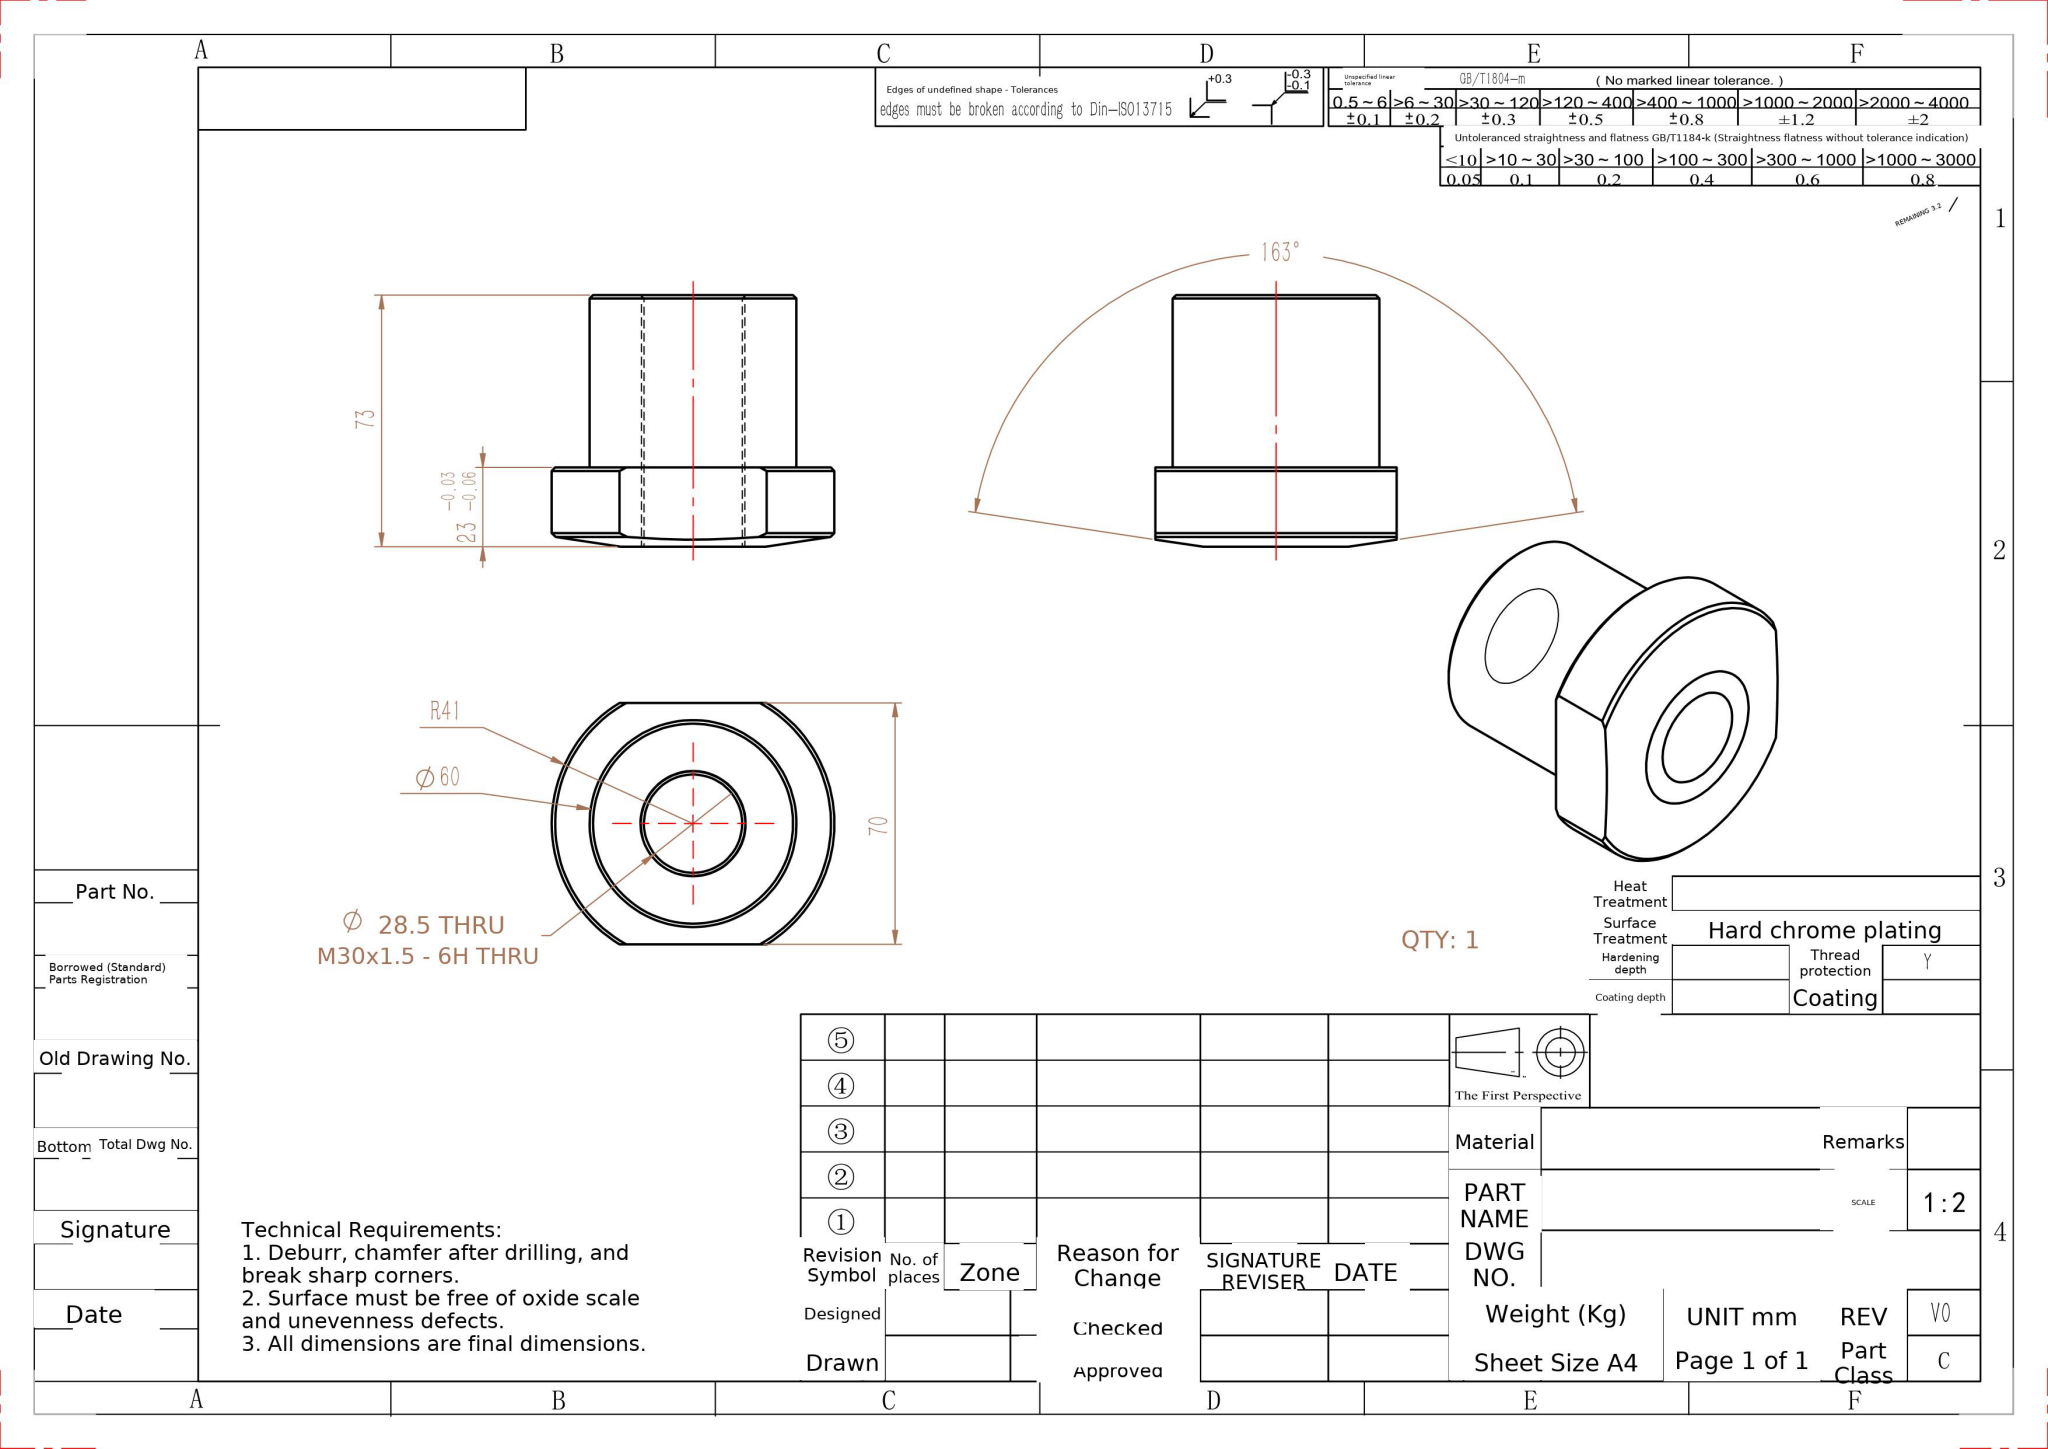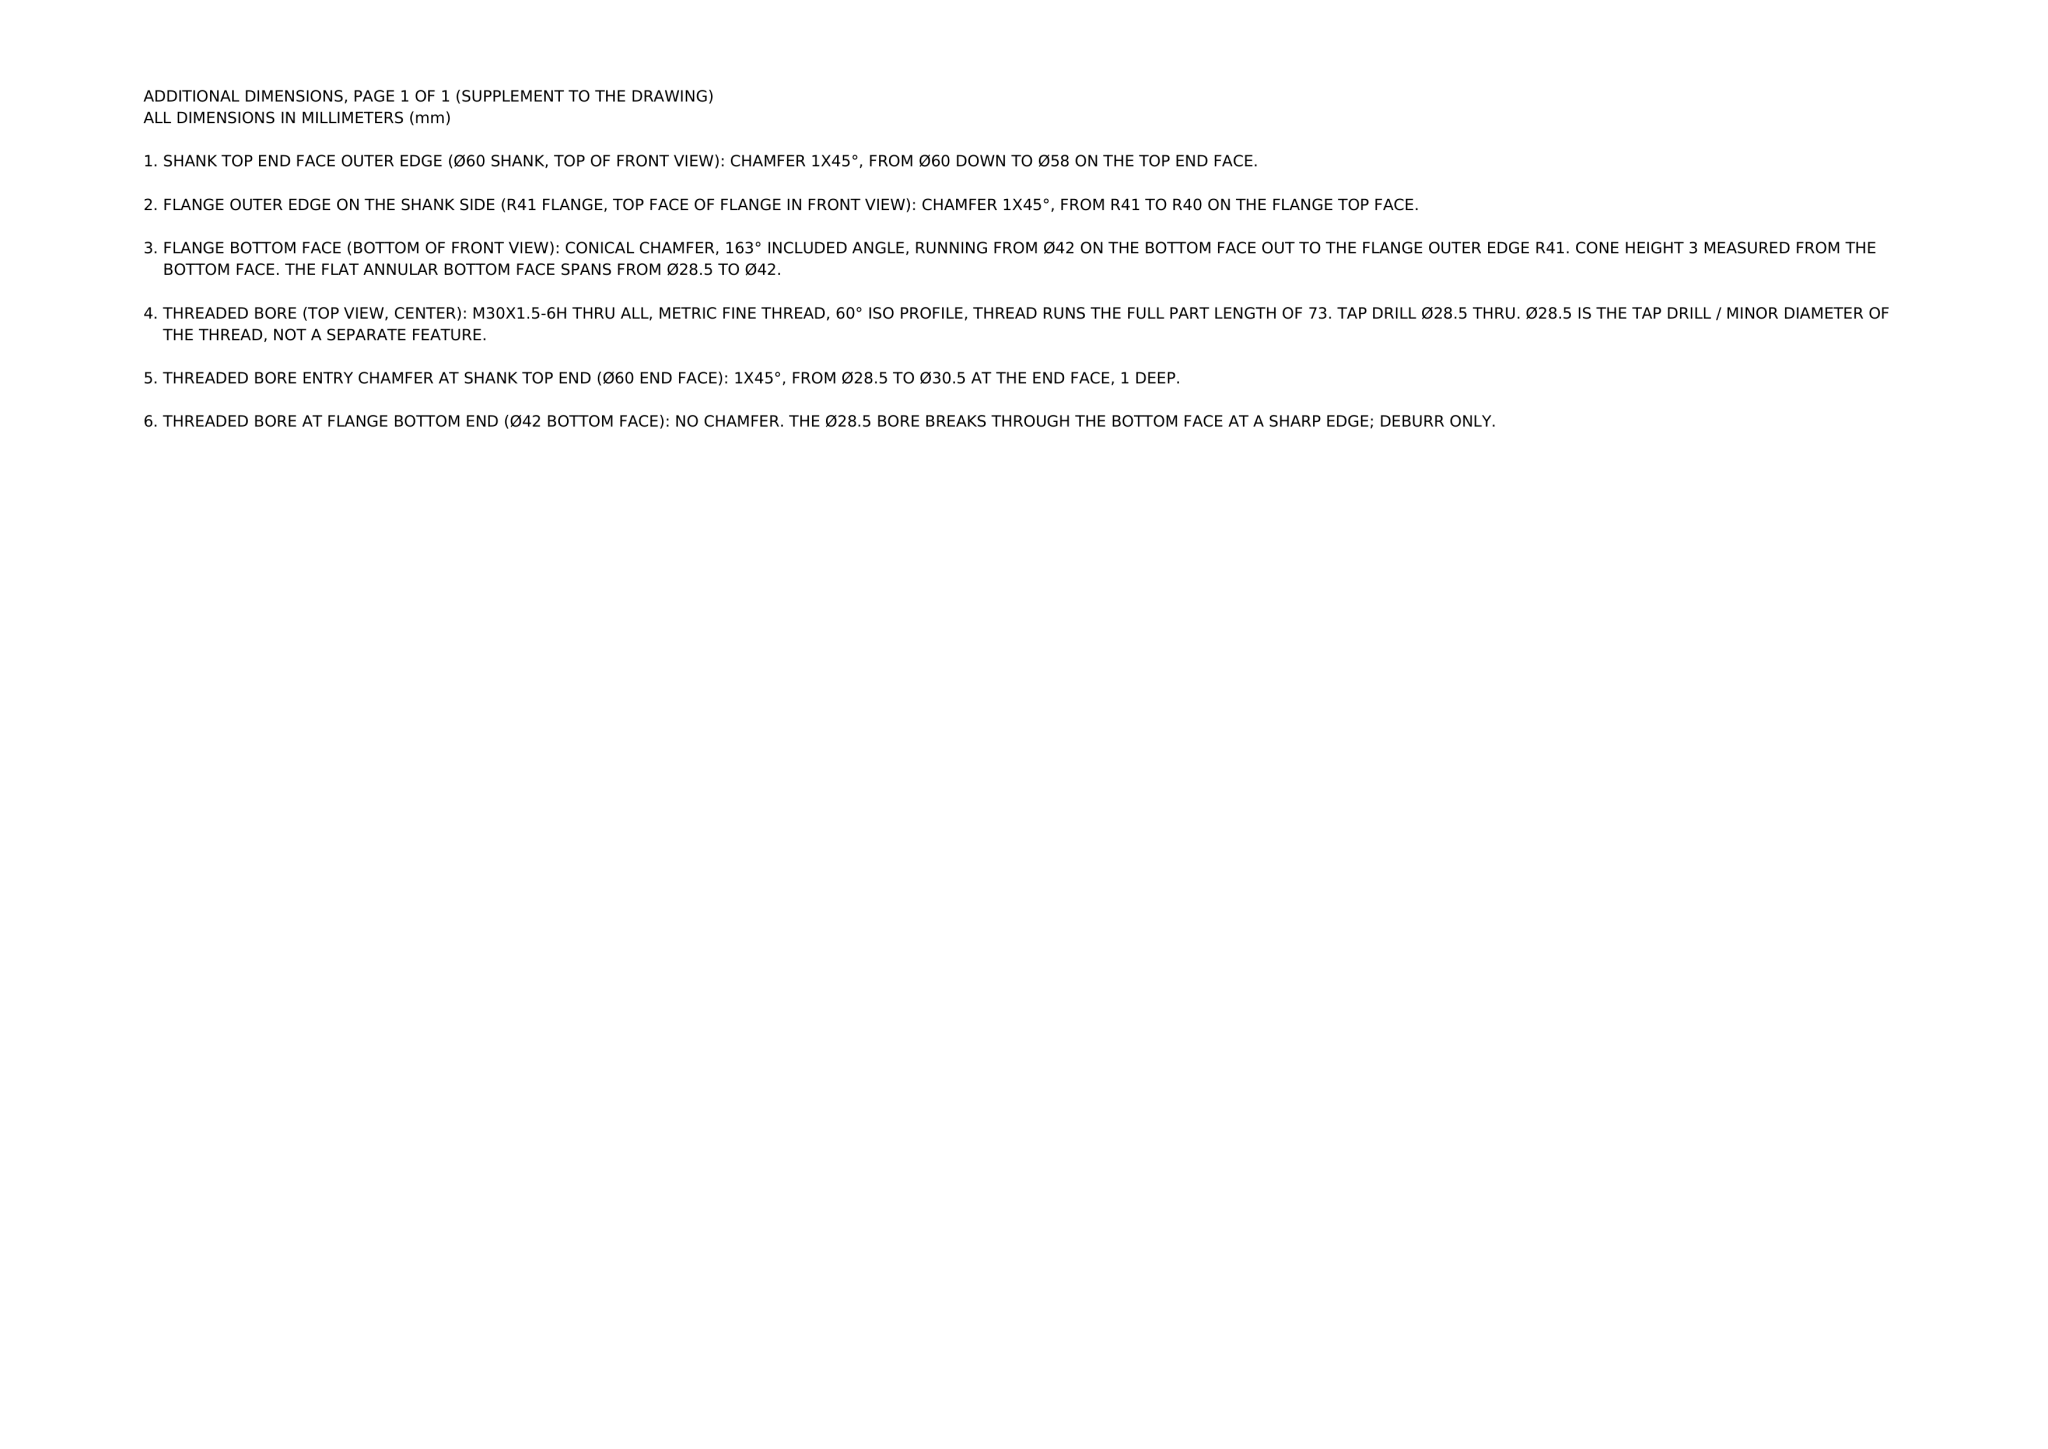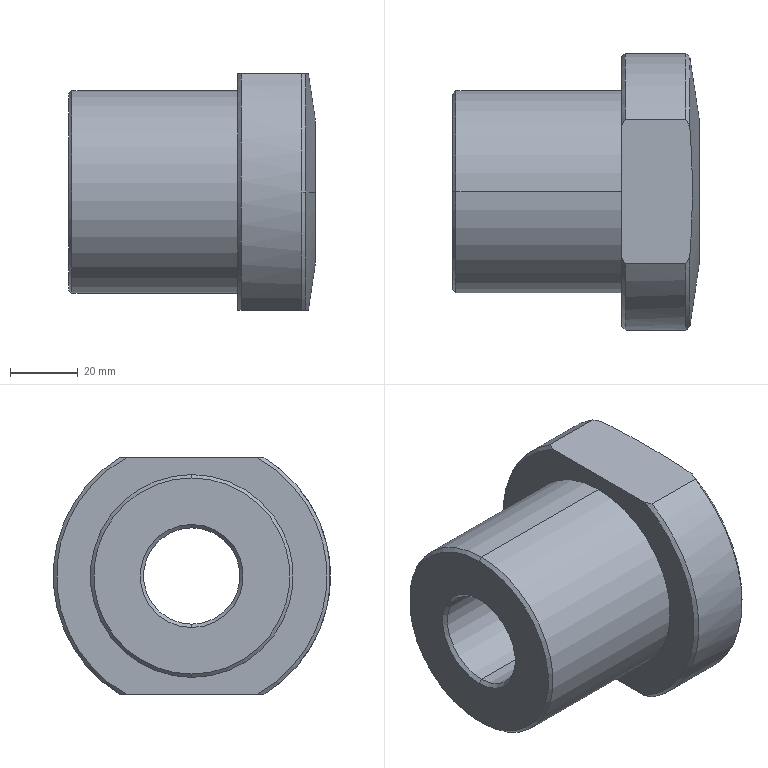Part | NX | mm | 1 solid | 22 faces | box 73 x 82 x 70 mm | volume 202408 mm3 | cone 11 | cylinder 6 | plane 5 | commonest cylinder face diameters 28.5 x2 60 x2 82 x2
STEP:
#1=CARTESIAN_POINT('',(23.176,-39.824,0.));
#2=VERTEX_POINT('',#1);
#3=CARTESIAN_POINT('',(23.176,-18.998,-35.));
#4=VERTEX_POINT('',#3);
#5=CARTESIAN_POINT('',(23.176,0.,0.));
#6=DIRECTION('',(1.,0.,0.));
#7=DIRECTION('',(-0.,1.,0.));
#8=AXIS2_PLACEMENT_3D('',#5,#6,#7);
#9=CIRCLE('',#8,39.824);
#10=EDGE_CURVE('',#2,#4,#9,.T.);
#11=ORIENTED_EDGE('',*,*,#10,.F.);
#12=CARTESIAN_POINT('',(22.,-41.,0.));
#13=VERTEX_POINT('',#12);
#14=CARTESIAN_POINT('',(23.176,-39.824,0.));
#15=DIRECTION('',(-0.7071,-0.7071,0.));
#16=VECTOR('',#15,1000.);
#17=LINE('',#14,#16);
#18=EDGE_CURVE('',#2,#13,#17,.T.);
#19=ORIENTED_EDGE('',*,*,#18,.T.);
#20=CARTESIAN_POINT('',(22.,-21.354,-35.));
#21=VERTEX_POINT('',#20);
#22=CARTESIAN_POINT('',(22.,0.,0.));
#23=DIRECTION('',(-1.,-0.,0.));
#24=DIRECTION('',(-0.,1.,0.));
#25=AXIS2_PLACEMENT_3D('',#22,#23,#24);
#26=CIRCLE('',#25,41.);
#27=EDGE_CURVE('',#21,#13,#26,.T.);
#28=ORIENTED_EDGE('',*,*,#27,.F.);
#29=CARTESIAN_POINT('',(23.176,-18.998,-35.));
#30=CARTESIAN_POINT('',(22.798,-19.79,-35.));
#31=CARTESIAN_POINT('',(22.406,-20.575,-35.));
#32=CARTESIAN_POINT('',(22.,-21.354,-35.));
#33=B_SPLINE_CURVE_WITH_KNOTS('',3,(#29,#30,#31,#32),.UNSPECIFIED.,.F.,.F.,(4,4),(0.,0.002634),.UNSPECIFIED.);
#34=EDGE_CURVE('',#4,#21,#33,.T.);
#35=ORIENTED_EDGE('',*,*,#34,.F.);
#36=EDGE_LOOP('',(#11,#19,#28,#35));
#37=FACE_OUTER_BOUND('',#36,.T.);
#38=CARTESIAN_POINT('',(23.176,0.,0.));
#39=DIRECTION('',(-1.,-0.,0.));
#40=DIRECTION('',(0.,-1.,0.));
#41=AXIS2_PLACEMENT_3D('',#38,#39,#40);
#42=CONICAL_SURFACE('',#41,39.824,0.7854);
#43=ADVANCED_FACE('',(#37),#42,.T.);
#44=CARTESIAN_POINT('',(-47.,0.,29.));
#45=VERTEX_POINT('',#44);
#46=CARTESIAN_POINT('',(-47.,0.,-29.));
#47=VERTEX_POINT('',#46);
#48=CARTESIAN_POINT('',(-47.,0.,0.));
#49=DIRECTION('',(-1.,0.,0.));
#50=DIRECTION('',(0.,0.,1.));
#51=AXIS2_PLACEMENT_3D('',#48,#49,#50);
#52=CIRCLE('',#51,29.);
#53=EDGE_CURVE('',#45,#47,#52,.T.);
#54=ORIENTED_EDGE('',*,*,#53,.F.);
#55=CARTESIAN_POINT('',(-46.,0.,30.));
#56=VERTEX_POINT('',#55);
#57=CARTESIAN_POINT('',(-47.,0.,29.));
#58=DIRECTION('',(0.7071,0.,0.7071));
#59=VECTOR('',#58,1000.);
#60=LINE('',#57,#59);
#61=EDGE_CURVE('',#45,#56,#60,.T.);
#62=ORIENTED_EDGE('',*,*,#61,.T.);
#63=CARTESIAN_POINT('',(-46.,0.,-30.));
#64=VERTEX_POINT('',#63);
#65=CARTESIAN_POINT('',(-46.,0.,0.));
#66=DIRECTION('',(1.,0.,0.));
#67=DIRECTION('',(0.,0.,1.));
#68=AXIS2_PLACEMENT_3D('',#65,#66,#67);
#69=CIRCLE('',#68,30.);
#70=EDGE_CURVE('',#64,#56,#69,.T.);
#71=ORIENTED_EDGE('',*,*,#70,.F.);
#72=CARTESIAN_POINT('',(-47.,0.,-29.));
#73=DIRECTION('',(0.7071,0.,-0.7071));
#74=VECTOR('',#73,1000.);
#75=LINE('',#72,#74);
#76=EDGE_CURVE('',#47,#64,#75,.T.);
#77=ORIENTED_EDGE('',*,*,#76,.F.);
#78=EDGE_LOOP('',(#54,#62,#71,#77));
#79=FACE_OUTER_BOUND('',#78,.T.);
#80=CARTESIAN_POINT('',(-47.,0.,0.));
#81=DIRECTION('',(1.,0.,0.));
#82=DIRECTION('',(0.,0.,-1.));
#83=AXIS2_PLACEMENT_3D('',#80,#81,#82);
#84=CONICAL_SURFACE('',#83,29.,0.7854);
#85=ADVANCED_FACE('',(#79),#84,.T.);
#86=CARTESIAN_POINT('',(-46.,0.,-14.25));
#87=VERTEX_POINT('',#86);
#88=CARTESIAN_POINT('',(-46.,0.,14.25));
#89=VERTEX_POINT('',#88);
#90=CARTESIAN_POINT('',(-46.,0.,0.));
#91=DIRECTION('',(-1.,0.,0.));
#92=DIRECTION('',(0.,0.,1.));
#93=AXIS2_PLACEMENT_3D('',#90,#91,#92);
#94=CIRCLE('',#93,14.25);
#95=EDGE_CURVE('',#87,#89,#94,.T.);
#96=ORIENTED_EDGE('',*,*,#95,.F.);
#97=CARTESIAN_POINT('',(-47.,0.,-15.25));
#98=VERTEX_POINT('',#97);
#99=CARTESIAN_POINT('',(-46.,0.,-14.25));
#100=DIRECTION('',(-0.7071,0.,-0.7071));
#101=VECTOR('',#100,1000.);
#102=LINE('',#99,#101);
#103=EDGE_CURVE('',#87,#98,#102,.T.);
#104=ORIENTED_EDGE('',*,*,#103,.T.);
#105=CARTESIAN_POINT('',(-47.,0.,15.25));
#106=VERTEX_POINT('',#105);
#107=CARTESIAN_POINT('',(-47.,0.,0.));
#108=DIRECTION('',(1.,0.,0.));
#109=DIRECTION('',(0.,0.,1.));
#110=AXIS2_PLACEMENT_3D('',#107,#108,#109);
#111=CIRCLE('',#110,15.25);
#112=EDGE_CURVE('',#106,#98,#111,.T.);
#113=ORIENTED_EDGE('',*,*,#112,.F.);
#114=CARTESIAN_POINT('',(-46.,0.,14.25));
#115=DIRECTION('',(-0.7071,0.,0.7071));
#116=VECTOR('',#115,1000.);
#117=LINE('',#114,#116);
#118=EDGE_CURVE('',#89,#106,#117,.T.);
#119=ORIENTED_EDGE('',*,*,#118,.F.);
#120=EDGE_LOOP('',(#96,#104,#113,#119));
#121=FACE_OUTER_BOUND('',#120,.T.);
#122=CARTESIAN_POINT('',(-46.,0.,0.));
#123=DIRECTION('',(-1.,0.,0.));
#124=DIRECTION('',(0.,0.,1.));
#125=AXIS2_PLACEMENT_3D('',#122,#123,#124);
#126=CONICAL_SURFACE('',#125,14.25,0.7854);
#127=ADVANCED_FACE('',(#121),#126,.F.);
#128=CARTESIAN_POINT('',(26.,0.,-14.25));
#129=VERTEX_POINT('',#128);
#130=CARTESIAN_POINT('',(26.,0.,14.25));
#131=VERTEX_POINT('',#130);
#132=CARTESIAN_POINT('',(26.,0.,0.));
#133=DIRECTION('',(-1.,0.,0.));
#134=DIRECTION('',(0.,0.,1.));
#135=AXIS2_PLACEMENT_3D('',#132,#133,#134);
#136=CIRCLE('',#135,14.25);
#137=EDGE_CURVE('',#129,#131,#136,.T.);
#138=ORIENTED_EDGE('',*,*,#137,.F.);
#139=CARTESIAN_POINT('',(-47.,0.,-14.25));
#140=DIRECTION('',(-1.,0.,0.));
#141=VECTOR('',#140,1000.);
#142=LINE('',#139,#141);
#143=EDGE_CURVE('',#129,#87,#142,.T.);
#144=ORIENTED_EDGE('',*,*,#143,.T.);
#145=ORIENTED_EDGE('',*,*,#95,.T.);
#146=CARTESIAN_POINT('',(-47.,0.,14.25));
#147=DIRECTION('',(-1.,0.,0.));
#148=VECTOR('',#147,1000.);
#149=LINE('',#146,#148);
#150=EDGE_CURVE('',#131,#89,#149,.T.);
#151=ORIENTED_EDGE('',*,*,#150,.F.);
#152=EDGE_LOOP('',(#138,#144,#145,#151));
#153=FACE_OUTER_BOUND('',#152,.T.);
#154=CARTESIAN_POINT('',(-47.,0.,0.));
#155=DIRECTION('',(-1.,0.,0.));
#156=DIRECTION('',(0.,0.,1.));
#157=AXIS2_PLACEMENT_3D('',#154,#155,#156);
#158=CYLINDRICAL_SURFACE('',#157,14.25);
#159=ADVANCED_FACE('',(#153),#158,.F.);
#160=ORIENTED_EDGE('',*,*,#70,.T.);
#161=CARTESIAN_POINT('',(3.,0.,30.));
#162=VERTEX_POINT('',#161);
#163=CARTESIAN_POINT('',(-47.,0.,30.));
#164=DIRECTION('',(1.,0.,0.));
#165=VECTOR('',#164,1000.);
#166=LINE('',#163,#165);
#167=EDGE_CURVE('',#56,#162,#166,.T.);
#168=ORIENTED_EDGE('',*,*,#167,.T.);
#169=CARTESIAN_POINT('',(3.,0.,-30.));
#170=VERTEX_POINT('',#169);
#171=CARTESIAN_POINT('',(3.,0.,0.));
#172=DIRECTION('',(-1.,0.,0.));
#173=DIRECTION('',(0.,0.,1.));
#174=AXIS2_PLACEMENT_3D('',#171,#172,#173);
#175=CIRCLE('',#174,30.);
#176=EDGE_CURVE('',#162,#170,#175,.T.);
#177=ORIENTED_EDGE('',*,*,#176,.T.);
#178=CARTESIAN_POINT('',(-47.,0.,-30.));
#179=DIRECTION('',(1.,0.,0.));
#180=VECTOR('',#179,1000.);
#181=LINE('',#178,#180);
#182=EDGE_CURVE('',#64,#170,#181,.T.);
#183=ORIENTED_EDGE('',*,*,#182,.F.);
#184=EDGE_LOOP('',(#160,#168,#177,#183));
#185=FACE_OUTER_BOUND('',#184,.T.);
#186=CARTESIAN_POINT('',(-47.,0.,0.));
#187=DIRECTION('',(1.,0.,0.));
#188=DIRECTION('',(0.,0.,-1.));
#189=AXIS2_PLACEMENT_3D('',#186,#187,#188);
#190=CYLINDRICAL_SURFACE('',#189,30.);
#191=ADVANCED_FACE('',(#185),#190,.T.);
#192=CARTESIAN_POINT('',(26.,21.,0.));
#193=VERTEX_POINT('',#192);
#194=CARTESIAN_POINT('',(26.,-21.,0.));
#195=VERTEX_POINT('',#194);
#196=CARTESIAN_POINT('',(26.,0.,0.));
#197=DIRECTION('',(1.,0.,0.));
#198=DIRECTION('',(-0.,1.,0.));
#199=AXIS2_PLACEMENT_3D('',#196,#197,#198);
#200=CIRCLE('',#199,21.);
#201=EDGE_CURVE('',#193,#195,#200,.T.);
#202=ORIENTED_EDGE('',*,*,#201,.F.);
#203=CARTESIAN_POINT('',(23.176,39.824,0.));
#204=VERTEX_POINT('',#203);
#205=CARTESIAN_POINT('',(26.,21.,0.));
#206=DIRECTION('',(-0.1483,0.9889,0.));
#207=VECTOR('',#206,1000.);
#208=LINE('',#205,#207);
#209=EDGE_CURVE('',#193,#204,#208,.T.);
#210=ORIENTED_EDGE('',*,*,#209,.T.);
#211=CARTESIAN_POINT('',(23.176,18.998,35.));
#212=VERTEX_POINT('',#211);
#213=CARTESIAN_POINT('',(23.176,0.,0.));
#214=DIRECTION('',(1.,0.,0.));
#215=DIRECTION('',(-0.,1.,0.));
#216=AXIS2_PLACEMENT_3D('',#213,#214,#215);
#217=CIRCLE('',#216,39.824);
#218=EDGE_CURVE('',#204,#212,#217,.T.);
#219=ORIENTED_EDGE('',*,*,#218,.T.);
#220=CARTESIAN_POINT('',(23.176,-18.998,35.));
#221=VERTEX_POINT('',#220);
#222=CARTESIAN_POINT('',(23.176,18.998,35.));
#223=CARTESIAN_POINT('',(23.402,15.846,35.));
#224=CARTESIAN_POINT('',(23.584,12.691,35.));
#225=CARTESIAN_POINT('',(23.833,6.372,35.));
#226=CARTESIAN_POINT('',(23.899,3.208,35.));
#227=CARTESIAN_POINT('',(23.901,-3.129,35.));
#228=CARTESIAN_POINT('',(23.835,-6.303,35.));
#229=CARTESIAN_POINT('',(23.586,-12.659,35.));
#230=CARTESIAN_POINT('',(23.403,-15.83,35.));
#231=CARTESIAN_POINT('',(23.176,-18.998,35.));
#232=B_SPLINE_CURVE_WITH_KNOTS('',3,(#222,#223,#224,#225,#226,#227,#228,#229,#230,#231),.UNSPECIFIED.,.F.,.F.,(4,2,2,2,4),(0.04542,0.0549,0.06438,0.07386,0.08334),.UNSPECIFIED.);
#233=EDGE_CURVE('',#212,#221,#232,.T.);
#234=ORIENTED_EDGE('',*,*,#233,.T.);
#235=CARTESIAN_POINT('',(23.176,0.,0.));
#236=DIRECTION('',(1.,0.,0.));
#237=DIRECTION('',(-0.,1.,0.));
#238=AXIS2_PLACEMENT_3D('',#235,#236,#237);
#239=CIRCLE('',#238,39.824);
#240=EDGE_CURVE('',#221,#2,#239,.T.);
#241=ORIENTED_EDGE('',*,*,#240,.T.);
#242=CARTESIAN_POINT('',(26.,-21.,0.));
#243=DIRECTION('',(-0.1483,-0.9889,0.));
#244=VECTOR('',#243,1000.);
#245=LINE('',#242,#244);
#246=EDGE_CURVE('',#195,#2,#245,.T.);
#247=ORIENTED_EDGE('',*,*,#246,.F.);
#248=EDGE_LOOP('',(#202,#210,#219,#234,#241,#247));
#249=FACE_OUTER_BOUND('',#248,.T.);
#250=CARTESIAN_POINT('',(26.,0.,0.));
#251=DIRECTION('',(-1.,-0.,0.));
#252=DIRECTION('',(0.,-1.,0.));
#253=AXIS2_PLACEMENT_3D('',#250,#251,#252);
#254=CONICAL_SURFACE('',#253,21.,1.422);
#255=ADVANCED_FACE('',(#249),#254,.T.);
#256=CARTESIAN_POINT('',(22.,21.354,35.));
#257=VERTEX_POINT('',#256);
#258=CARTESIAN_POINT('',(4.,21.354,35.));
#259=VERTEX_POINT('',#258);
#260=CARTESIAN_POINT('',(141.966,21.354,35.));
#261=DIRECTION('',(-1.,0.,0.));
#262=VECTOR('',#261,1000.);
#263=LINE('',#260,#262);
#264=EDGE_CURVE('',#257,#259,#263,.T.);
#265=ORIENTED_EDGE('',*,*,#264,.F.);
#266=CARTESIAN_POINT('',(22.,21.354,-35.));
#267=VERTEX_POINT('',#266);
#268=CARTESIAN_POINT('',(22.,0.,0.));
#269=DIRECTION('',(-1.,-0.,0.));
#270=DIRECTION('',(-0.,1.,0.));
#271=AXIS2_PLACEMENT_3D('',#268,#269,#270);
#272=CIRCLE('',#271,41.);
#273=EDGE_CURVE('',#257,#267,#272,.T.);
#274=ORIENTED_EDGE('',*,*,#273,.T.);
#275=CARTESIAN_POINT('',(4.,21.354,-35.));
#276=VERTEX_POINT('',#275);
#277=CARTESIAN_POINT('',(141.966,21.354,-35.));
#278=DIRECTION('',(1.,0.,0.));
#279=VECTOR('',#278,1000.);
#280=LINE('',#277,#279);
#281=EDGE_CURVE('',#276,#267,#280,.T.);
#282=ORIENTED_EDGE('',*,*,#281,.F.);
#283=CARTESIAN_POINT('',(4.,0.,0.));
#284=DIRECTION('',(1.,0.,0.));
#285=DIRECTION('',(0.,-0.,1.));
#286=AXIS2_PLACEMENT_3D('',#283,#284,#285);
#287=CIRCLE('',#286,41.);
#288=EDGE_CURVE('',#276,#259,#287,.T.);
#289=ORIENTED_EDGE('',*,*,#288,.T.);
#290=EDGE_LOOP('',(#265,#274,#282,#289));
#291=FACE_OUTER_BOUND('',#290,.T.);
#292=CARTESIAN_POINT('',(141.966,0.,0.));
#293=DIRECTION('',(-1.,0.,0.));
#294=DIRECTION('',(0.,0.,1.));
#295=AXIS2_PLACEMENT_3D('',#292,#293,#294);
#296=CYLINDRICAL_SURFACE('',#295,41.);
#297=ADVANCED_FACE('',(#291),#296,.T.);
#298=CARTESIAN_POINT('',(4.,-21.354,-35.));
#299=VERTEX_POINT('',#298);
#300=CARTESIAN_POINT('',(141.966,-21.354,-35.));
#301=DIRECTION('',(-1.,0.,0.));
#302=VECTOR('',#301,1000.);
#303=LINE('',#300,#302);
#304=EDGE_CURVE('',#21,#299,#303,.T.);
#305=ORIENTED_EDGE('',*,*,#304,.F.);
#306=ORIENTED_EDGE('',*,*,#27,.T.);
#307=CARTESIAN_POINT('',(22.,-21.354,35.));
#308=VERTEX_POINT('',#307);
#309=CARTESIAN_POINT('',(22.,0.,0.));
#310=DIRECTION('',(-1.,-0.,0.));
#311=DIRECTION('',(-0.,1.,0.));
#312=AXIS2_PLACEMENT_3D('',#309,#310,#311);
#313=CIRCLE('',#312,41.);
#314=EDGE_CURVE('',#13,#308,#313,.T.);
#315=ORIENTED_EDGE('',*,*,#314,.T.);
#316=CARTESIAN_POINT('',(4.,-21.354,35.));
#317=VERTEX_POINT('',#316);
#318=CARTESIAN_POINT('',(141.966,-21.354,35.));
#319=DIRECTION('',(1.,0.,0.));
#320=VECTOR('',#319,1000.);
#321=LINE('',#318,#320);
#322=EDGE_CURVE('',#317,#308,#321,.T.);
#323=ORIENTED_EDGE('',*,*,#322,.F.);
#324=CARTESIAN_POINT('',(4.,0.,0.));
#325=DIRECTION('',(1.,0.,0.));
#326=DIRECTION('',(0.,0.,1.));
#327=AXIS2_PLACEMENT_3D('',#324,#325,#326);
#328=CIRCLE('',#327,41.);
#329=EDGE_CURVE('',#317,#299,#328,.T.);
#330=ORIENTED_EDGE('',*,*,#329,.T.);
#331=EDGE_LOOP('',(#305,#306,#315,#323,#330));
#332=FACE_OUTER_BOUND('',#331,.T.);
#333=CARTESIAN_POINT('',(141.966,0.,0.));
#334=DIRECTION('',(-1.,0.,0.));
#335=DIRECTION('',(0.,0.,1.));
#336=AXIS2_PLACEMENT_3D('',#333,#334,#335);
#337=CYLINDRICAL_SURFACE('',#336,41.);
#338=ADVANCED_FACE('',(#332),#337,.T.);
#339=ORIENTED_EDGE('',*,*,#233,.F.);
#340=CARTESIAN_POINT('',(23.176,18.998,35.));
#341=CARTESIAN_POINT('',(22.798,19.79,35.));
#342=CARTESIAN_POINT('',(22.406,20.575,35.));
#343=CARTESIAN_POINT('',(22.,21.354,35.));
#344=B_SPLINE_CURVE_WITH_KNOTS('',3,(#340,#341,#342,#343),.UNSPECIFIED.,.F.,.F.,(4,4),(0.,0.002634),.UNSPECIFIED.);
#345=EDGE_CURVE('',#212,#257,#344,.T.);
#346=ORIENTED_EDGE('',*,*,#345,.T.);
#347=ORIENTED_EDGE('',*,*,#264,.T.);
#348=CARTESIAN_POINT('',(3.,19.365,35.));
#349=VERTEX_POINT('',#348);
#350=CARTESIAN_POINT('',(4.,21.354,35.));
#351=CARTESIAN_POINT('',(3.657,20.696,35.));
#352=CARTESIAN_POINT('',(3.323,20.033,35.));
#353=CARTESIAN_POINT('',(3.,19.365,35.));
#354=B_SPLINE_CURVE_WITH_KNOTS('',3,(#350,#351,#352,#353),.UNSPECIFIED.,.F.,.F.,(4,4),(0.,0.002226),.UNSPECIFIED.);
#355=EDGE_CURVE('',#259,#349,#354,.T.);
#356=ORIENTED_EDGE('',*,*,#355,.T.);
#357=CARTESIAN_POINT('',(3.,-19.365,35.));
#358=VERTEX_POINT('',#357);
#359=CARTESIAN_POINT('',(3.,45.286,35.));
#360=DIRECTION('',(0.,-1.,0.));
#361=VECTOR('',#360,1000.);
#362=LINE('',#359,#361);
#363=EDGE_CURVE('',#349,#358,#362,.T.);
#364=ORIENTED_EDGE('',*,*,#363,.T.);
#365=CARTESIAN_POINT('',(3.,-19.365,35.));
#366=CARTESIAN_POINT('',(3.323,-20.033,35.));
#367=CARTESIAN_POINT('',(3.657,-20.696,35.));
#368=CARTESIAN_POINT('',(4.,-21.354,35.));
#369=B_SPLINE_CURVE_WITH_KNOTS('',3,(#365,#366,#367,#368),.UNSPECIFIED.,.F.,.F.,(4,4),(0.,0.002226),.UNSPECIFIED.);
#370=EDGE_CURVE('',#358,#317,#369,.T.);
#371=ORIENTED_EDGE('',*,*,#370,.T.);
#372=ORIENTED_EDGE('',*,*,#322,.T.);
#373=CARTESIAN_POINT('',(22.,-21.354,35.));
#374=CARTESIAN_POINT('',(22.406,-20.575,35.));
#375=CARTESIAN_POINT('',(22.798,-19.79,35.));
#376=CARTESIAN_POINT('',(23.176,-18.998,35.));
#377=B_SPLINE_CURVE_WITH_KNOTS('',3,(#373,#374,#375,#376),.UNSPECIFIED.,.F.,.F.,(4,4),(0.,0.002634),.UNSPECIFIED.);
#378=EDGE_CURVE('',#308,#221,#377,.T.);
#379=ORIENTED_EDGE('',*,*,#378,.T.);
#380=EDGE_LOOP('',(#339,#346,#347,#356,#364,#371,#372,#379));
#381=FACE_OUTER_BOUND('',#380,.T.);
#382=CARTESIAN_POINT('',(26.,45.286,35.));
#383=DIRECTION('',(0.,-0.,-1.));
#384=DIRECTION('',(0.,1.,-0.));
#385=AXIS2_PLACEMENT_3D('',#382,#383,#384);
#386=PLANE('',#385);
#387=ADVANCED_FACE('',(#381),#386,.F.);
#388=ORIENTED_EDGE('',*,*,#281,.T.);
#389=CARTESIAN_POINT('',(23.176,18.998,-35.));
#390=VERTEX_POINT('',#389);
#391=CARTESIAN_POINT('',(22.,21.354,-35.));
#392=CARTESIAN_POINT('',(22.406,20.575,-35.));
#393=CARTESIAN_POINT('',(22.798,19.79,-35.));
#394=CARTESIAN_POINT('',(23.176,18.998,-35.));
#395=B_SPLINE_CURVE_WITH_KNOTS('',3,(#391,#392,#393,#394),.UNSPECIFIED.,.F.,.F.,(4,4),(0.,0.002634),.UNSPECIFIED.);
#396=EDGE_CURVE('',#267,#390,#395,.T.);
#397=ORIENTED_EDGE('',*,*,#396,.T.);
#398=CARTESIAN_POINT('',(23.176,-18.998,-35.));
#399=CARTESIAN_POINT('',(23.402,-15.846,-35.));
#400=CARTESIAN_POINT('',(23.584,-12.691,-35.));
#401=CARTESIAN_POINT('',(23.833,-6.372,-35.));
#402=CARTESIAN_POINT('',(23.899,-3.208,-35.));
#403=CARTESIAN_POINT('',(23.901,3.129,-35.));
#404=CARTESIAN_POINT('',(23.835,6.303,-35.));
#405=CARTESIAN_POINT('',(23.586,12.659,-35.));
#406=CARTESIAN_POINT('',(23.403,15.83,-35.));
#407=CARTESIAN_POINT('',(23.176,18.998,-35.));
#408=B_SPLINE_CURVE_WITH_KNOTS('',3,(#398,#399,#400,#401,#402,#403,#404,#405,#406,#407),.UNSPECIFIED.,.F.,.F.,(4,2,2,2,4),(0.04542,0.0549,0.06438,0.07386,0.08334),.UNSPECIFIED.);
#409=EDGE_CURVE('',#4,#390,#408,.T.);
#410=ORIENTED_EDGE('',*,*,#409,.F.);
#411=ORIENTED_EDGE('',*,*,#34,.T.);
#412=ORIENTED_EDGE('',*,*,#304,.T.);
#413=CARTESIAN_POINT('',(3.,-19.365,-35.));
#414=VERTEX_POINT('',#413);
#415=CARTESIAN_POINT('',(4.,-21.354,-35.));
#416=CARTESIAN_POINT('',(3.657,-20.696,-35.));
#417=CARTESIAN_POINT('',(3.323,-20.033,-35.));
#418=CARTESIAN_POINT('',(3.,-19.365,-35.));
#419=B_SPLINE_CURVE_WITH_KNOTS('',3,(#415,#416,#417,#418),.UNSPECIFIED.,.F.,.F.,(4,4),(0.,0.002226),.UNSPECIFIED.);
#420=EDGE_CURVE('',#299,#414,#419,.T.);
#421=ORIENTED_EDGE('',*,*,#420,.T.);
#422=CARTESIAN_POINT('',(3.,19.365,-35.));
#423=VERTEX_POINT('',#422);
#424=CARTESIAN_POINT('',(3.,43.028,-35.));
#425=DIRECTION('',(0.,1.,-0.));
#426=VECTOR('',#425,1000.);
#427=LINE('',#424,#426);
#428=EDGE_CURVE('',#414,#423,#427,.T.);
#429=ORIENTED_EDGE('',*,*,#428,.T.);
#430=CARTESIAN_POINT('',(3.,19.365,-35.));
#431=CARTESIAN_POINT('',(3.323,20.033,-35.));
#432=CARTESIAN_POINT('',(3.657,20.696,-35.));
#433=CARTESIAN_POINT('',(4.,21.354,-35.));
#434=B_SPLINE_CURVE_WITH_KNOTS('',3,(#430,#431,#432,#433),.UNSPECIFIED.,.F.,.F.,(4,4),(0.,0.002226),.UNSPECIFIED.);
#435=EDGE_CURVE('',#423,#276,#434,.T.);
#436=ORIENTED_EDGE('',*,*,#435,.T.);
#437=EDGE_LOOP('',(#388,#397,#410,#411,#412,#421,#429,#436));
#438=FACE_OUTER_BOUND('',#437,.T.);
#439=CARTESIAN_POINT('',(26.,43.028,-35.));
#440=DIRECTION('',(0.,0.,1.));
#441=DIRECTION('',(0.,-1.,0.));
#442=AXIS2_PLACEMENT_3D('',#439,#440,#441);
#443=PLANE('',#442);
#444=ADVANCED_FACE('',(#438),#443,.F.);
#445=CARTESIAN_POINT('',(3.,0.,0.));
#446=DIRECTION('',(-1.,0.,0.));
#447=DIRECTION('',(0.,0.,1.));
#448=AXIS2_PLACEMENT_3D('',#445,#446,#447);
#449=CIRCLE('',#448,30.);
#450=EDGE_CURVE('',#170,#162,#449,.T.);
#451=ORIENTED_EDGE('',*,*,#450,.F.);
#452=ORIENTED_EDGE('',*,*,#176,.F.);
#453=EDGE_LOOP('',(#451,#452));
#454=FACE_BOUND('',#453,.T.);
#455=ORIENTED_EDGE('',*,*,#428,.F.);
#456=CARTESIAN_POINT('',(3.,0.,0.));
#457=DIRECTION('',(-1.,0.,0.));
#458=DIRECTION('',(0.,0.,1.));
#459=AXIS2_PLACEMENT_3D('',#456,#457,#458);
#460=CIRCLE('',#459,40.);
#461=EDGE_CURVE('',#414,#358,#460,.T.);
#462=ORIENTED_EDGE('',*,*,#461,.T.);
#463=ORIENTED_EDGE('',*,*,#363,.F.);
#464=CARTESIAN_POINT('',(3.,0.,0.));
#465=DIRECTION('',(-1.,0.,0.));
#466=DIRECTION('',(0.,0.,1.));
#467=AXIS2_PLACEMENT_3D('',#464,#465,#466);
#468=CIRCLE('',#467,40.);
#469=EDGE_CURVE('',#349,#423,#468,.T.);
#470=ORIENTED_EDGE('',*,*,#469,.T.);
#471=EDGE_LOOP('',(#455,#462,#463,#470));
#472=FACE_OUTER_BOUND('',#471,.T.);
#473=CARTESIAN_POINT('',(3.,26.5,0.));
#474=DIRECTION('',(-1.,0.,0.));
#475=DIRECTION('',(0.,0.,1.));
#476=AXIS2_PLACEMENT_3D('',#473,#474,#475);
#477=PLANE('',#476);
#478=ADVANCED_FACE('',(#454,#472),#477,.T.);
#479=ORIENTED_EDGE('',*,*,#209,.F.);
#480=CARTESIAN_POINT('',(26.,0.,0.));
#481=DIRECTION('',(1.,0.,0.));
#482=DIRECTION('',(-0.,1.,0.));
#483=AXIS2_PLACEMENT_3D('',#480,#481,#482);
#484=CIRCLE('',#483,21.);
#485=EDGE_CURVE('',#195,#193,#484,.T.);
#486=ORIENTED_EDGE('',*,*,#485,.F.);
#487=ORIENTED_EDGE('',*,*,#246,.T.);
#488=ORIENTED_EDGE('',*,*,#10,.T.);
#489=ORIENTED_EDGE('',*,*,#409,.T.);
#490=CARTESIAN_POINT('',(23.176,0.,0.));
#491=DIRECTION('',(1.,0.,0.));
#492=DIRECTION('',(-0.,1.,0.));
#493=AXIS2_PLACEMENT_3D('',#490,#491,#492);
#494=CIRCLE('',#493,39.824);
#495=EDGE_CURVE('',#390,#204,#494,.T.);
#496=ORIENTED_EDGE('',*,*,#495,.T.);
#497=EDGE_LOOP('',(#479,#486,#487,#488,#489,#496));
#498=FACE_OUTER_BOUND('',#497,.T.);
#499=CARTESIAN_POINT('',(26.,0.,0.));
#500=DIRECTION('',(-1.,-0.,0.));
#501=DIRECTION('',(0.,-1.,0.));
#502=AXIS2_PLACEMENT_3D('',#499,#500,#501);
#503=CONICAL_SURFACE('',#502,21.,1.422);
#504=ADVANCED_FACE('',(#498),#503,.T.);
#505=CARTESIAN_POINT('',(26.,0.,0.));
#506=DIRECTION('',(-1.,0.,0.));
#507=DIRECTION('',(0.,0.,1.));
#508=AXIS2_PLACEMENT_3D('',#505,#506,#507);
#509=CIRCLE('',#508,14.25);
#510=EDGE_CURVE('',#131,#129,#509,.T.);
#511=ORIENTED_EDGE('',*,*,#510,.T.);
#512=ORIENTED_EDGE('',*,*,#137,.T.);
#513=EDGE_LOOP('',(#511,#512));
#514=FACE_BOUND('',#513,.T.);
#515=ORIENTED_EDGE('',*,*,#485,.T.);
#516=ORIENTED_EDGE('',*,*,#201,.T.);
#517=EDGE_LOOP('',(#515,#516));
#518=FACE_OUTER_BOUND('',#517,.T.);
#519=CARTESIAN_POINT('',(26.,13.,0.));
#520=DIRECTION('',(1.,0.,0.));
#521=DIRECTION('',(0.,0.,-1.));
#522=AXIS2_PLACEMENT_3D('',#519,#520,#521);
#523=PLANE('',#522);
#524=ADVANCED_FACE('',(#514,#518),#523,.T.);
#525=ORIENTED_EDGE('',*,*,#167,.F.);
#526=CARTESIAN_POINT('',(-46.,0.,0.));
#527=DIRECTION('',(1.,0.,0.));
#528=DIRECTION('',(0.,0.,1.));
#529=AXIS2_PLACEMENT_3D('',#526,#527,#528);
#530=CIRCLE('',#529,30.);
#531=EDGE_CURVE('',#56,#64,#530,.T.);
#532=ORIENTED_EDGE('',*,*,#531,.T.);
#533=ORIENTED_EDGE('',*,*,#182,.T.);
#534=ORIENTED_EDGE('',*,*,#450,.T.);
#535=EDGE_LOOP('',(#525,#532,#533,#534));
#536=FACE_OUTER_BOUND('',#535,.T.);
#537=CARTESIAN_POINT('',(-47.,0.,0.));
#538=DIRECTION('',(1.,0.,0.));
#539=DIRECTION('',(0.,0.,-1.));
#540=AXIS2_PLACEMENT_3D('',#537,#538,#539);
#541=CYLINDRICAL_SURFACE('',#540,30.);
#542=ADVANCED_FACE('',(#536),#541,.T.);
#543=ORIENTED_EDGE('',*,*,#112,.T.);
#544=CARTESIAN_POINT('',(-47.,0.,0.));
#545=DIRECTION('',(1.,0.,0.));
#546=DIRECTION('',(0.,0.,1.));
#547=AXIS2_PLACEMENT_3D('',#544,#545,#546);
#548=CIRCLE('',#547,15.25);
#549=EDGE_CURVE('',#98,#106,#548,.T.);
#550=ORIENTED_EDGE('',*,*,#549,.T.);
#551=EDGE_LOOP('',(#543,#550));
#552=FACE_BOUND('',#551,.T.);
#553=CARTESIAN_POINT('',(-47.,0.,0.));
#554=DIRECTION('',(-1.,0.,0.));
#555=DIRECTION('',(0.,0.,1.));
#556=AXIS2_PLACEMENT_3D('',#553,#554,#555);
#557=CIRCLE('',#556,29.);
#558=EDGE_CURVE('',#47,#45,#557,.T.);
#559=ORIENTED_EDGE('',*,*,#558,.T.);
#560=ORIENTED_EDGE('',*,*,#53,.T.);
#561=EDGE_LOOP('',(#559,#560));
#562=FACE_OUTER_BOUND('',#561,.T.);
#563=CARTESIAN_POINT('',(-47.,0.,0.));
#564=DIRECTION('',(-1.,0.,0.));
#565=DIRECTION('',(0.,0.,1.));
#566=AXIS2_PLACEMENT_3D('',#563,#564,#565);
#567=PLANE('',#566);
#568=ADVANCED_FACE('',(#552,#562),#567,.T.);
#569=ORIENTED_EDGE('',*,*,#143,.F.);
#570=ORIENTED_EDGE('',*,*,#510,.F.);
#571=ORIENTED_EDGE('',*,*,#150,.T.);
#572=CARTESIAN_POINT('',(-46.,0.,0.));
#573=DIRECTION('',(-1.,0.,0.));
#574=DIRECTION('',(0.,0.,1.));
#575=AXIS2_PLACEMENT_3D('',#572,#573,#574);
#576=CIRCLE('',#575,14.25);
#577=EDGE_CURVE('',#89,#87,#576,.T.);
#578=ORIENTED_EDGE('',*,*,#577,.T.);
#579=EDGE_LOOP('',(#569,#570,#571,#578));
#580=FACE_OUTER_BOUND('',#579,.T.);
#581=CARTESIAN_POINT('',(-47.,0.,0.));
#582=DIRECTION('',(-1.,0.,0.));
#583=DIRECTION('',(0.,0.,1.));
#584=AXIS2_PLACEMENT_3D('',#581,#582,#583);
#585=CYLINDRICAL_SURFACE('',#584,14.25);
#586=ADVANCED_FACE('',(#580),#585,.F.);
#587=ORIENTED_EDGE('',*,*,#103,.F.);
#588=ORIENTED_EDGE('',*,*,#577,.F.);
#589=ORIENTED_EDGE('',*,*,#118,.T.);
#590=ORIENTED_EDGE('',*,*,#549,.F.);
#591=EDGE_LOOP('',(#587,#588,#589,#590));
#592=FACE_OUTER_BOUND('',#591,.T.);
#593=CARTESIAN_POINT('',(-46.,0.,0.));
#594=DIRECTION('',(-1.,0.,0.));
#595=DIRECTION('',(0.,0.,1.));
#596=AXIS2_PLACEMENT_3D('',#593,#594,#595);
#597=CONICAL_SURFACE('',#596,14.25,0.7854);
#598=ADVANCED_FACE('',(#592),#597,.F.);
#599=ORIENTED_EDGE('',*,*,#61,.F.);
#600=ORIENTED_EDGE('',*,*,#558,.F.);
#601=ORIENTED_EDGE('',*,*,#76,.T.);
#602=ORIENTED_EDGE('',*,*,#531,.F.);
#603=EDGE_LOOP('',(#599,#600,#601,#602));
#604=FACE_OUTER_BOUND('',#603,.T.);
#605=CARTESIAN_POINT('',(-47.,0.,0.));
#606=DIRECTION('',(1.,0.,0.));
#607=DIRECTION('',(0.,0.,-1.));
#608=AXIS2_PLACEMENT_3D('',#605,#606,#607);
#609=CONICAL_SURFACE('',#608,29.,0.7854);
#610=ADVANCED_FACE('',(#604),#609,.T.);
#611=ORIENTED_EDGE('',*,*,#396,.F.);
#612=ORIENTED_EDGE('',*,*,#273,.F.);
#613=ORIENTED_EDGE('',*,*,#345,.F.);
#614=ORIENTED_EDGE('',*,*,#218,.F.);
#615=ORIENTED_EDGE('',*,*,#495,.F.);
#616=EDGE_LOOP('',(#611,#612,#613,#614,#615));
#617=FACE_OUTER_BOUND('',#616,.T.);
#618=CARTESIAN_POINT('',(23.176,0.,0.));
#619=DIRECTION('',(-1.,-0.,0.));
#620=DIRECTION('',(0.,-1.,0.));
#621=AXIS2_PLACEMENT_3D('',#618,#619,#620);
#622=CONICAL_SURFACE('',#621,39.824,0.7854);
#623=ADVANCED_FACE('',(#617),#622,.T.);
#624=ORIENTED_EDGE('',*,*,#18,.F.);
#625=ORIENTED_EDGE('',*,*,#240,.F.);
#626=ORIENTED_EDGE('',*,*,#378,.F.);
#627=ORIENTED_EDGE('',*,*,#314,.F.);
#628=EDGE_LOOP('',(#624,#625,#626,#627));
#629=FACE_OUTER_BOUND('',#628,.T.);
#630=CARTESIAN_POINT('',(23.176,0.,0.));
#631=DIRECTION('',(-1.,-0.,0.));
#632=DIRECTION('',(0.,-1.,0.));
#633=AXIS2_PLACEMENT_3D('',#630,#631,#632);
#634=CONICAL_SURFACE('',#633,39.824,0.7854);
#635=ADVANCED_FACE('',(#629),#634,.T.);
#636=ORIENTED_EDGE('',*,*,#420,.F.);
#637=ORIENTED_EDGE('',*,*,#329,.F.);
#638=ORIENTED_EDGE('',*,*,#370,.F.);
#639=ORIENTED_EDGE('',*,*,#461,.F.);
#640=EDGE_LOOP('',(#636,#637,#638,#639));
#641=FACE_OUTER_BOUND('',#640,.T.);
#642=CARTESIAN_POINT('',(3.,0.,0.));
#643=DIRECTION('',(1.,0.,0.));
#644=DIRECTION('',(0.,0.,-1.));
#645=AXIS2_PLACEMENT_3D('',#642,#643,#644);
#646=CONICAL_SURFACE('',#645,40.,0.7854);
#647=ADVANCED_FACE('',(#641),#646,.T.);
#648=ORIENTED_EDGE('',*,*,#355,.F.);
#649=ORIENTED_EDGE('',*,*,#288,.F.);
#650=ORIENTED_EDGE('',*,*,#435,.F.);
#651=ORIENTED_EDGE('',*,*,#469,.F.);
#652=EDGE_LOOP('',(#648,#649,#650,#651));
#653=FACE_OUTER_BOUND('',#652,.T.);
#654=CARTESIAN_POINT('',(3.,0.,0.));
#655=DIRECTION('',(1.,0.,0.));
#656=DIRECTION('',(0.,0.,-1.));
#657=AXIS2_PLACEMENT_3D('',#654,#655,#656);
#658=CONICAL_SURFACE('',#657,40.,0.7854);
#659=ADVANCED_FACE('',(#653),#658,.T.);
#660=CLOSED_SHELL('',(#43,#85,#127,#159,#191,#255,#297,#338,#387,#444,#478,#504,#524,#542,#568,#586,#598,#610,#623,#635,#647,#659));
#661=MANIFOLD_SOLID_BREP('',#660);
#662=CARTESIAN_POINT('',(0.,0.,0.));
#663=DIRECTION('',(0.,0.,1.));
#664=DIRECTION('',(1.,0.,0.));
#665=AXIS2_PLACEMENT_3D('',#662,#663,#664);
#666=(LENGTH_UNIT()NAMED_UNIT(*)SI_UNIT(.MILLI.,.METRE.));
#667=UNCERTAINTY_MEASURE_WITH_UNIT(LENGTH_MEASURE(0.00001),#666,'','');
#668=(NAMED_UNIT(*)PLANE_ANGLE_UNIT()SI_UNIT($,.RADIAN.));
#669=(NAMED_UNIT(*)SI_UNIT($,.STERADIAN.)SOLID_ANGLE_UNIT());
#670=(GEOMETRIC_REPRESENTATION_CONTEXT(3)GLOBAL_UNCERTAINTY_ASSIGNED_CONTEXT((#667))GLOBAL_UNIT_ASSIGNED_CONTEXT((#666,#668,#669))REPRESENTATION_CONTEXT('',''));
#671=ADVANCED_BREP_SHAPE_REPRESENTATION('',(#661,#665),#670);
#672=COLOUR_RGB('',0.7922,0.8196,0.9333);
#673=FILL_AREA_STYLE_COLOUR('',#672);
#674=FILL_AREA_STYLE('',(#673));
#675=SURFACE_STYLE_FILL_AREA(#674);
#676=SURFACE_SIDE_STYLE('',(#675));
#677=SURFACE_STYLE_USAGE(.BOTH.,#676);
#678=PRESENTATION_STYLE_ASSIGNMENT((#677));
#679=STYLED_ITEM('',(#678),#661);
#680=(LENGTH_UNIT()NAMED_UNIT(*)SI_UNIT(.MILLI.,.METRE.));
#681=UNCERTAINTY_MEASURE_WITH_UNIT(LENGTH_MEASURE(0.00001),#680,'','');
#682=(NAMED_UNIT(*)PLANE_ANGLE_UNIT()SI_UNIT($,.RADIAN.));
#683=(NAMED_UNIT(*)SI_UNIT($,.STERADIAN.)SOLID_ANGLE_UNIT());
#684=(GEOMETRIC_REPRESENTATION_CONTEXT(3)GLOBAL_UNCERTAINTY_ASSIGNED_CONTEXT((#681))GLOBAL_UNIT_ASSIGNED_CONTEXT((#680,#682,#683))REPRESENTATION_CONTEXT('',''));
#685=MECHANICAL_DESIGN_GEOMETRIC_PRESENTATION_REPRESENTATION('',(#679),#684);
#686=PRESENTATION_LAYER_ASSIGNMENT('','',(#679));